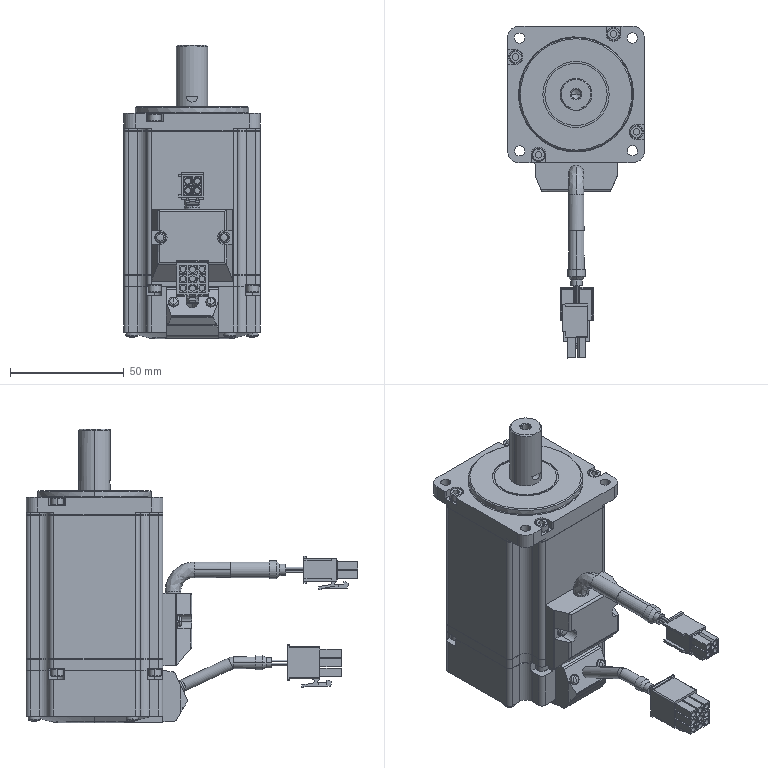Component | SolidWorks | Q1-A12-S21-Q1A.SLDASQ-1_Q1-QSQF042L1U2-2 | 7 solids | 967 faces | volume 347365 mm3 | plane 562 | cylinder 304 | cone 63 | spline 34 | torus 4 | commonest cylinder face diameters 1 x35 4 x33 6 x29 2.6 x26 3.92 x20 5.5 x16 8 x16 2 x13